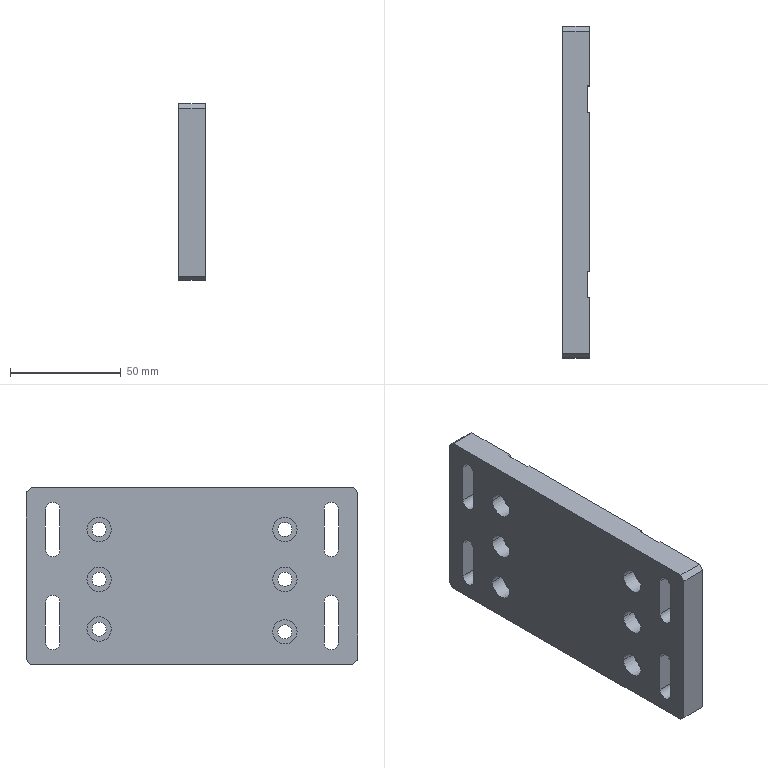Component | SolidWorks | Part7RobotArmBase-Copy-1 | 1 solid | 64 faces | box 12 x 150 x 80 mm | volume 129933 mm3 | cylinder 32 | plane 32 | commonest cylinder face diameters 11 x12 6.4 x12 6.6 x8 | material Plain Carbon Steel
build123d program:
from build123d import *
from OCP.BRepFilletAPI import BRepFilletAPI_MakeChamfer

# Parameters (mm, degrees)
SKETCH1_W                                         = 150
SKETCH1_H                                         = 80
BOSS_EXTRUDE1_DEPTH                               = 12
SKETCH2_W                                         = 12
SKETCH2_H                                         = 80
CUT_EXTRUDE1_DEPTH                                = 1
CHAMFER1_SIZE                                     = 2
CHAMFER1_SIZE2                                    = 2.384
HOLE_SIZE_ACCORDING_TO_TYPE_1_OF_HEXA_D           = 6.4
HOLE_SIZE_ACCORDING_TO_TYPE_1_OF_HEXA_DEPTH       = 15
HOLE_SIZE_ACCORDING_TO_TYPE_1_OF_HEXA_CBORE_D     = 11
HOLE_SIZE_ACCORDING_TO_TYPE_1_OF_HEXA_CBORE_DEPTH = 6.8
HOLE_SIZE_ACCORDING_TO_TYPE_1_OF_HEXA_TIP         = 1.923
CUT_EXTRUDE2_DEPTH                                = 86.843


with BuildPart() as part:
    # Sketch1 → Boss-Extrude1 (new body)
    with BuildSketch(Plane.XY):
        Rectangle(SKETCH1_W, SKETCH1_H)
    extrude(amount=BOSS_EXTRUDE1_DEPTH)

    # Sketch2 → Cut-Extrude1 (cut)
    with BuildSketch(Plane.XY.offset(12)):
        with Locations((-42, 0)):
            Rectangle(SKETCH2_W, SKETCH2_H)
        with Locations((42, 0)):
            Rectangle(SKETCH2_W, SKETCH2_H)
    extrude(amount=-CUT_EXTRUDE1_DEPTH, mode=Mode.SUBTRACT)

    # Chamfer1: one chamfer whose edges measure the first distance from different faces: ONE call of the kernel's chamfer builder (chamfer() names one face for all edges)
    chamfer1_edges_1 = [part.edges().sort_by_distance(p)[0] for p in [
        (75, -40, 6),
    ]]
    chamfer1_side_1 = [part.faces().sort_by_distance(p)[0] for p in [
        (0, -40, 5.926),
    ]]
    chamfer1_edges_2 = [part.edges().sort_by_distance(p)[0] for p in [
        (-75, -40, 6),
    ]]
    chamfer1_side_2 = [part.faces().sort_by_distance(p)[0] for p in [
        (-75, 0, 6),
    ]]
    chamfer1_edges_3 = [part.edges().sort_by_distance(p)[0] for p in [
        (-75, 40, 6),
    ]]
    chamfer1_side_3 = [part.faces().sort_by_distance(p)[0] for p in [
        (0, 40, 5.926),
    ]]
    chamfer1_edges_4 = [part.edges().sort_by_distance(p)[0] for p in [
        (75, 40, 6),
    ]]
    chamfer1_side_4 = [part.faces().sort_by_distance(p)[0] for p in [
        (75, 0, 6),
    ]]
    chamfer1 = BRepFilletAPI_MakeChamfer(part.part.solid().wrapped)
    for e in chamfer1_edges_1:
        chamfer1.Add(CHAMFER1_SIZE, CHAMFER1_SIZE2, e.wrapped, chamfer1_side_1[0].wrapped)  # the first distance lies on this face
    for e in chamfer1_edges_2:
        chamfer1.Add(CHAMFER1_SIZE, CHAMFER1_SIZE2, e.wrapped, chamfer1_side_2[0].wrapped)  # the first distance lies on this face
    for e in chamfer1_edges_3:
        chamfer1.Add(CHAMFER1_SIZE, CHAMFER1_SIZE2, e.wrapped, chamfer1_side_3[0].wrapped)  # the first distance lies on this face
    for e in chamfer1_edges_4:
        chamfer1.Add(CHAMFER1_SIZE, CHAMFER1_SIZE2, e.wrapped, chamfer1_side_4[0].wrapped)  # the first distance lies on this face
    add(Compound.cast(chamfer1.Shape()), mode=Mode.REPLACE)

    # Hole Size _ according to_ Type 1 of Hexa
    with Locations(Plane(origin=(0, 0, 0), x_dir=(-1, 0, 0), z_dir=(0, 0, -1))):
        with Locations((-42, 21), (-42, -1.5), (-42, -24), (42, 21), (42, -1.5), (42, -25.25)):
            CounterBoreHole(HOLE_SIZE_ACCORDING_TO_TYPE_1_OF_HEXA_D / 2, HOLE_SIZE_ACCORDING_TO_TYPE_1_OF_HEXA_CBORE_D / 2, HOLE_SIZE_ACCORDING_TO_TYPE_1_OF_HEXA_CBORE_DEPTH, depth=HOLE_SIZE_ACCORDING_TO_TYPE_1_OF_HEXA_DEPTH)
            with Locations((0, 0, -(HOLE_SIZE_ACCORDING_TO_TYPE_1_OF_HEXA_DEPTH + HOLE_SIZE_ACCORDING_TO_TYPE_1_OF_HEXA_TIP / 2))):  # 118° drill point
                Cone(0, HOLE_SIZE_ACCORDING_TO_TYPE_1_OF_HEXA_D / 2, HOLE_SIZE_ACCORDING_TO_TYPE_1_OF_HEXA_TIP, mode=Mode.SUBTRACT)

    # Sketch5 → Cut-Extrude2 (cut, through all)
    with BuildSketch(Plane.XY.offset(12)):
        with BuildLine():
            Line((-59.7, 30), (-59.7, 12))
            ThreePointArc((-59.7, 12), (-63, 8.7), (-66.3, 12))
            Line((-66.3, 12), (-66.3, 30))
            ThreePointArc((-66.3, 30), (-63, 33.3), (-59.7, 30))
        make_face()
        with BuildLine():
            Line((59.7, 30), (59.7, 12))
            ThreePointArc((59.7, 12), (63, 8.7), (66.3, 12))
            Line((66.3, 12), (66.3, 30))
            ThreePointArc((66.3, 30), (63, 33.3), (59.7, 30))
        make_face()
        with BuildLine():
            Line((-59.7, -30), (-59.7, -12))
            ThreePointArc((-59.7, -12), (-63, -8.7), (-66.3, -12))
            Line((-66.3, -12), (-66.3, -30))
            ThreePointArc((-66.3, -30), (-63, -33.3), (-59.7, -30))
        make_face()
        with BuildLine():
            Line((59.7, -30), (59.7, -12))
            ThreePointArc((59.7, -12), (63, -8.7), (66.3, -12))
            Line((66.3, -12), (66.3, -30))
            ThreePointArc((66.3, -30), (63, -33.3), (59.7, -30))
        make_face()
    extrude(amount=-CUT_EXTRUDE2_DEPTH, mode=Mode.SUBTRACT)


solid = part.part

# Placed as in the assembly
solid = solid.moved(Location((-338.522, 19.945, 113.051), (90, 90, 0)))